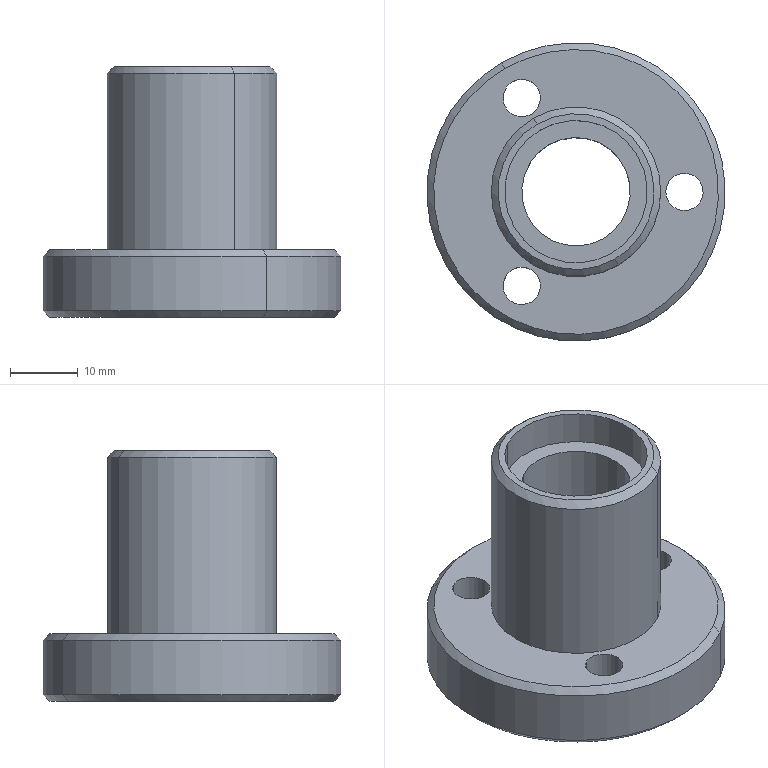Component | SolidWorks | JYTBJ-HeaderPlateFlangeSeatB-1 | 1 solid | 36 faces | box 44 x 44 x 37 mm | volume 17743 mm3 | cylinder 22 | plane 8 | cone 6 | commonest cylinder face diameters 10 x6 5.5 x6 21 x4 25 x2 16 x2 44 x2
STEP:
#1=COLOUR_RGB('',0.7922,0.8196,0.9333);
#2=FILL_AREA_STYLE_COLOUR('',#1);
#3=FILL_AREA_STYLE('',(#2));
#4=SURFACE_STYLE_FILL_AREA(#3);
#5=SURFACE_SIDE_STYLE('',(#4));
#6=SURFACE_STYLE_USAGE(.BOTH.,#5);
#7=PRESENTATION_STYLE_ASSIGNMENT((#6));
#8=CARTESIAN_POINT('',(-3.046,9.321,-0.03937));
#9=VERTEX_POINT('',#8);
#10=CARTESIAN_POINT('',(-2.594,8.536,-0.03937));
#11=VERTEX_POINT('',#10);
#12=CARTESIAN_POINT('',(-2.82,8.928,-0.03937));
#13=DIRECTION('',(0.,0.,1.));
#14=DIRECTION('',(-0.5,0.866,0.));
#15=AXIS2_PLACEMENT_3D('',#12,#13,#14);
#16=CIRCLE('',#15,0.4528);
#17=EDGE_CURVE('',#9,#11,#16,.T.);
#18=ORIENTED_EDGE('',*,*,#17,.F.);
#19=CARTESIAN_POINT('',(-3.066,9.355,-0.07874));
#20=VERTEX_POINT('',#19);
#21=CARTESIAN_POINT('',(-3.066,9.355,-0.07874));
#22=DIRECTION('',(-0.3536,0.6124,-0.7071));
#23=VECTOR('',#22,39.37);
#24=LINE('',#21,#23);
#25=EDGE_CURVE('',#9,#20,#24,.T.);
#26=ORIENTED_EDGE('',*,*,#25,.T.);
#27=CARTESIAN_POINT('',(-2.574,8.502,-0.07874));
#28=VERTEX_POINT('',#27);
#29=CARTESIAN_POINT('',(-2.82,8.928,-0.07874));
#30=DIRECTION('',(0.,0.,-1.));
#31=DIRECTION('',(-0.5,0.866,0.));
#32=AXIS2_PLACEMENT_3D('',#29,#30,#31);
#33=CIRCLE('',#32,0.4921);
#34=EDGE_CURVE('',#28,#20,#33,.T.);
#35=ORIENTED_EDGE('',*,*,#34,.F.);
#36=CARTESIAN_POINT('',(-2.574,8.502,-0.07874));
#37=DIRECTION('',(0.3536,-0.6124,-0.7071));
#38=VECTOR('',#37,39.37);
#39=LINE('',#36,#38);
#40=EDGE_CURVE('',#11,#28,#39,.T.);
#41=ORIENTED_EDGE('',*,*,#40,.F.);
#42=EDGE_LOOP('',(#18,#26,#35,#41));
#43=FACE_OUTER_BOUND('',#42,.T.);
#44=CARTESIAN_POINT('',(-2.82,8.928,-0.07874));
#45=DIRECTION('',(0.,0.,-1.));
#46=DIRECTION('',(0.5,-0.866,0.));
#47=AXIS2_PLACEMENT_3D('',#44,#45,#46);
#48=CONICAL_SURFACE('',#47,0.4921,0.7854);
#49=ADVANCED_FACE('',(#43),#48,.T.);
#50=CARTESIAN_POINT('',(-3.233,9.644,-1.102));
#51=VERTEX_POINT('',#50);
#52=CARTESIAN_POINT('',(-2.407,8.212,-1.102));
#53=VERTEX_POINT('',#52);
#54=CARTESIAN_POINT('',(-2.82,8.928,-1.102));
#55=DIRECTION('',(0.,0.,1.));
#56=DIRECTION('',(-0.5,0.866,0.));
#57=AXIS2_PLACEMENT_3D('',#54,#55,#56);
#58=CIRCLE('',#57,0.8268);
#59=EDGE_CURVE('',#51,#53,#58,.T.);
#60=ORIENTED_EDGE('',*,*,#59,.F.);
#61=CARTESIAN_POINT('',(-3.253,9.679,-1.142));
#62=VERTEX_POINT('',#61);
#63=CARTESIAN_POINT('',(-3.253,9.679,-1.142));
#64=DIRECTION('',(-0.3536,0.6124,-0.7071));
#65=VECTOR('',#64,39.37);
#66=LINE('',#63,#65);
#67=EDGE_CURVE('',#51,#62,#66,.T.);
#68=ORIENTED_EDGE('',*,*,#67,.T.);
#69=CARTESIAN_POINT('',(-2.387,8.178,-1.142));
#70=VERTEX_POINT('',#69);
#71=CARTESIAN_POINT('',(-2.82,8.928,-1.142));
#72=DIRECTION('',(0.,0.,-1.));
#73=DIRECTION('',(-0.5,0.866,0.));
#74=AXIS2_PLACEMENT_3D('',#71,#72,#73);
#75=CIRCLE('',#74,0.8661);
#76=EDGE_CURVE('',#70,#62,#75,.T.);
#77=ORIENTED_EDGE('',*,*,#76,.F.);
#78=CARTESIAN_POINT('',(-2.387,8.178,-1.142));
#79=DIRECTION('',(0.3536,-0.6124,-0.7071));
#80=VECTOR('',#79,39.37);
#81=LINE('',#78,#80);
#82=EDGE_CURVE('',#53,#70,#81,.T.);
#83=ORIENTED_EDGE('',*,*,#82,.F.);
#84=EDGE_LOOP('',(#60,#68,#77,#83));
#85=FACE_OUTER_BOUND('',#84,.T.);
#86=CARTESIAN_POINT('',(-2.82,8.928,-1.142));
#87=DIRECTION('',(0.,0.,-1.));
#88=DIRECTION('',(0.5,-0.866,0.));
#89=AXIS2_PLACEMENT_3D('',#86,#87,#88);
#90=CONICAL_SURFACE('',#89,0.8661,0.7854);
#91=ADVANCED_FACE('',(#85),#90,.T.);
#92=CARTESIAN_POINT('',(-2.407,8.212,-1.496));
#93=VERTEX_POINT('',#92);
#94=CARTESIAN_POINT('',(-3.233,8.212,-1.496));
#95=VERTEX_POINT('',#94);
#96=CARTESIAN_POINT('',(-2.82,8.928,-1.496));
#97=DIRECTION('',(0.,0.,-1.));
#98=DIRECTION('',(0.5,-0.866,0.));
#99=AXIS2_PLACEMENT_3D('',#96,#97,#98);
#100=CIRCLE('',#99,0.8268);
#101=EDGE_CURVE('',#93,#95,#100,.T.);
#102=ORIENTED_EDGE('',*,*,#101,.F.);
#103=CARTESIAN_POINT('',(-2.387,8.178,-1.457));
#104=VERTEX_POINT('',#103);
#105=CARTESIAN_POINT('',(-2.407,8.212,-1.496));
#106=DIRECTION('',(0.3536,-0.6124,0.7071));
#107=VECTOR('',#106,39.37);
#108=LINE('',#105,#107);
#109=EDGE_CURVE('',#93,#104,#108,.T.);
#110=ORIENTED_EDGE('',*,*,#109,.T.);
#111=CARTESIAN_POINT('',(-3.253,9.679,-1.457));
#112=VERTEX_POINT('',#111);
#113=CARTESIAN_POINT('',(-2.82,8.928,-1.457));
#114=DIRECTION('',(0.,0.,1.));
#115=DIRECTION('',(0.5,-0.866,0.));
#116=AXIS2_PLACEMENT_3D('',#113,#114,#115);
#117=CIRCLE('',#116,0.8661);
#118=EDGE_CURVE('',#112,#104,#117,.T.);
#119=ORIENTED_EDGE('',*,*,#118,.F.);
#120=CARTESIAN_POINT('',(-3.233,9.644,-1.496));
#121=VERTEX_POINT('',#120);
#122=CARTESIAN_POINT('',(-3.233,9.644,-1.496));
#123=DIRECTION('',(-0.3536,0.6124,0.7071));
#124=VECTOR('',#123,39.37);
#125=LINE('',#122,#124);
#126=EDGE_CURVE('',#121,#112,#125,.T.);
#127=ORIENTED_EDGE('',*,*,#126,.F.);
#128=CARTESIAN_POINT('',(-2.82,8.928,-1.496));
#129=DIRECTION('',(0.,0.,-1.));
#130=DIRECTION('',(0.5,-0.866,0.));
#131=AXIS2_PLACEMENT_3D('',#128,#129,#130);
#132=CIRCLE('',#131,0.8268);
#133=EDGE_CURVE('',#95,#121,#132,.T.);
#134=ORIENTED_EDGE('',*,*,#133,.F.);
#135=EDGE_LOOP('',(#102,#110,#119,#127,#134));
#136=FACE_OUTER_BOUND('',#135,.T.);
#137=CARTESIAN_POINT('',(-2.82,8.928,-1.496));
#138=DIRECTION('',(0.,0.,1.));
#139=DIRECTION('',(-0.5,0.866,0.));
#140=AXIS2_PLACEMENT_3D('',#137,#138,#139);
#141=CONICAL_SURFACE('',#140,0.8268,0.7854);
#142=ADVANCED_FACE('',(#136),#141,.T.);
#143=CARTESIAN_POINT('',(-3.233,8.553,-1.272));
#144=VERTEX_POINT('',#143);
#145=CARTESIAN_POINT('',(-3.036,8.212,-1.272));
#146=VERTEX_POINT('',#145);
#147=CARTESIAN_POINT('',(-3.135,8.383,-1.272));
#148=DIRECTION('',(0.,0.,-1.));
#149=DIRECTION('',(0.5,-0.866,0.));
#150=AXIS2_PLACEMENT_3D('',#147,#148,#149);
#151=CIRCLE('',#150,0.1969);
#152=EDGE_CURVE('',#144,#146,#151,.T.);
#153=ORIENTED_EDGE('',*,*,#152,.F.);
#154=CARTESIAN_POINT('',(-3.233,8.553,-1.496));
#155=VERTEX_POINT('',#154);
#156=CARTESIAN_POINT('',(-3.233,8.553,-1.496));
#157=DIRECTION('',(0.,0.,-1.));
#158=VECTOR('',#157,39.37);
#159=LINE('',#156,#158);
#160=EDGE_CURVE('',#144,#155,#159,.T.);
#161=ORIENTED_EDGE('',*,*,#160,.T.);
#162=CARTESIAN_POINT('',(-3.036,8.212,-1.496));
#163=VERTEX_POINT('',#162);
#164=CARTESIAN_POINT('',(-3.135,8.383,-1.496));
#165=DIRECTION('',(0.,0.,-1.));
#166=DIRECTION('',(0.5,-0.866,0.));
#167=AXIS2_PLACEMENT_3D('',#164,#165,#166);
#168=CIRCLE('',#167,0.1969);
#169=EDGE_CURVE('',#155,#163,#168,.T.);
#170=ORIENTED_EDGE('',*,*,#169,.T.);
#171=CARTESIAN_POINT('',(-3.036,8.212,-1.496));
#172=DIRECTION('',(0.,0.,-1.));
#173=VECTOR('',#172,39.37);
#174=LINE('',#171,#173);
#175=EDGE_CURVE('',#146,#163,#174,.T.);
#176=ORIENTED_EDGE('',*,*,#175,.F.);
#177=EDGE_LOOP('',(#153,#161,#170,#176));
#178=FACE_OUTER_BOUND('',#177,.T.);
#179=CARTESIAN_POINT('',(-3.135,8.383,-1.496));
#180=DIRECTION('',(0.,0.,-1.));
#181=DIRECTION('',(0.5,-0.866,0.));
#182=AXIS2_PLACEMENT_3D('',#179,#180,#181);
#183=CYLINDRICAL_SURFACE('',#182,0.1969);
#184=ADVANCED_FACE('',(#178),#183,.F.);
#185=CARTESIAN_POINT('',(-3.081,8.289,-1.102));
#186=VERTEX_POINT('',#185);
#187=CARTESIAN_POINT('',(-3.189,8.477,-1.102));
#188=VERTEX_POINT('',#187);
#189=CARTESIAN_POINT('',(-3.135,8.383,-1.102));
#190=DIRECTION('',(0.,0.,1.));
#191=DIRECTION('',(-0.5,0.866,0.));
#192=AXIS2_PLACEMENT_3D('',#189,#190,#191);
#193=CIRCLE('',#192,0.1083);
#194=EDGE_CURVE('',#186,#188,#193,.T.);
#195=ORIENTED_EDGE('',*,*,#194,.T.);
#196=CARTESIAN_POINT('',(-3.189,8.477,-1.272));
#197=VERTEX_POINT('',#196);
#198=CARTESIAN_POINT('',(-3.189,8.477,-1.496));
#199=DIRECTION('',(0.,0.,-1.));
#200=VECTOR('',#199,39.37);
#201=LINE('',#198,#200);
#202=EDGE_CURVE('',#188,#197,#201,.T.);
#203=ORIENTED_EDGE('',*,*,#202,.T.);
#204=CARTESIAN_POINT('',(-3.081,8.289,-1.272));
#205=VERTEX_POINT('',#204);
#206=CARTESIAN_POINT('',(-3.135,8.383,-1.272));
#207=DIRECTION('',(0.,0.,-1.));
#208=DIRECTION('',(0.5,-0.866,0.));
#209=AXIS2_PLACEMENT_3D('',#206,#207,#208);
#210=CIRCLE('',#209,0.1083);
#211=EDGE_CURVE('',#197,#205,#210,.T.);
#212=ORIENTED_EDGE('',*,*,#211,.T.);
#213=CARTESIAN_POINT('',(-3.081,8.289,-1.496));
#214=DIRECTION('',(0.,0.,-1.));
#215=VECTOR('',#214,39.37);
#216=LINE('',#213,#215);
#217=EDGE_CURVE('',#186,#205,#216,.T.);
#218=ORIENTED_EDGE('',*,*,#217,.F.);
#219=EDGE_LOOP('',(#195,#203,#212,#218));
#220=FACE_OUTER_BOUND('',#219,.T.);
#221=CARTESIAN_POINT('',(-3.135,8.383,-1.496));
#222=DIRECTION('',(0.,0.,-1.));
#223=DIRECTION('',(0.5,-0.866,0.));
#224=AXIS2_PLACEMENT_3D('',#221,#222,#223);
#225=CYLINDRICAL_SURFACE('',#224,0.1083);
#226=ADVANCED_FACE('',(#220),#225,.F.);
#227=CARTESIAN_POINT('',(-2.288,9.099,-1.272));
#228=VERTEX_POINT('',#227);
#229=CARTESIAN_POINT('',(-2.092,8.758,-1.272));
#230=VERTEX_POINT('',#229);
#231=CARTESIAN_POINT('',(-2.19,8.928,-1.272));
#232=DIRECTION('',(0.,0.,-1.));
#233=DIRECTION('',(0.5,-0.866,0.));
#234=AXIS2_PLACEMENT_3D('',#231,#232,#233);
#235=CIRCLE('',#234,0.1969);
#236=EDGE_CURVE('',#228,#230,#235,.T.);
#237=ORIENTED_EDGE('',*,*,#236,.F.);
#238=CARTESIAN_POINT('',(-2.288,9.099,-1.496));
#239=VERTEX_POINT('',#238);
#240=CARTESIAN_POINT('',(-2.288,9.099,-1.496));
#241=DIRECTION('',(0.,0.,-1.));
#242=VECTOR('',#241,39.37);
#243=LINE('',#240,#242);
#244=EDGE_CURVE('',#228,#239,#243,.T.);
#245=ORIENTED_EDGE('',*,*,#244,.T.);
#246=CARTESIAN_POINT('',(-1.993,8.928,-1.496));
#247=VERTEX_POINT('',#246);
#248=CARTESIAN_POINT('',(-2.19,8.928,-1.496));
#249=DIRECTION('',(0.,0.,-1.));
#250=DIRECTION('',(0.5,-0.866,0.));
#251=AXIS2_PLACEMENT_3D('',#248,#249,#250);
#252=CIRCLE('',#251,0.1969);
#253=EDGE_CURVE('',#239,#247,#252,.T.);
#254=ORIENTED_EDGE('',*,*,#253,.T.);
#255=CARTESIAN_POINT('',(-2.092,8.758,-1.496));
#256=VERTEX_POINT('',#255);
#257=CARTESIAN_POINT('',(-2.19,8.928,-1.496));
#258=DIRECTION('',(0.,0.,-1.));
#259=DIRECTION('',(0.5,-0.866,0.));
#260=AXIS2_PLACEMENT_3D('',#257,#258,#259);
#261=CIRCLE('',#260,0.1969);
#262=EDGE_CURVE('',#247,#256,#261,.T.);
#263=ORIENTED_EDGE('',*,*,#262,.T.);
#264=CARTESIAN_POINT('',(-2.092,8.758,-1.496));
#265=DIRECTION('',(0.,0.,-1.));
#266=VECTOR('',#265,39.37);
#267=LINE('',#264,#266);
#268=EDGE_CURVE('',#230,#256,#267,.T.);
#269=ORIENTED_EDGE('',*,*,#268,.F.);
#270=EDGE_LOOP('',(#237,#245,#254,#263,#269));
#271=FACE_OUTER_BOUND('',#270,.T.);
#272=CARTESIAN_POINT('',(-2.19,8.928,-1.496));
#273=DIRECTION('',(0.,0.,-1.));
#274=DIRECTION('',(0.5,-0.866,0.));
#275=AXIS2_PLACEMENT_3D('',#272,#273,#274);
#276=CYLINDRICAL_SURFACE('',#275,0.1969);
#277=ADVANCED_FACE('',(#271),#276,.F.);
#278=CARTESIAN_POINT('',(-2.136,8.835,-1.102));
#279=VERTEX_POINT('',#278);
#280=CARTESIAN_POINT('',(-2.244,9.022,-1.102));
#281=VERTEX_POINT('',#280);
#282=CARTESIAN_POINT('',(-2.19,8.928,-1.102));
#283=DIRECTION('',(0.,0.,1.));
#284=DIRECTION('',(-0.5,0.866,0.));
#285=AXIS2_PLACEMENT_3D('',#282,#283,#284);
#286=CIRCLE('',#285,0.1083);
#287=EDGE_CURVE('',#279,#281,#286,.T.);
#288=ORIENTED_EDGE('',*,*,#287,.T.);
#289=CARTESIAN_POINT('',(-2.244,9.022,-1.272));
#290=VERTEX_POINT('',#289);
#291=CARTESIAN_POINT('',(-2.244,9.022,-1.496));
#292=DIRECTION('',(0.,0.,-1.));
#293=VECTOR('',#292,39.37);
#294=LINE('',#291,#293);
#295=EDGE_CURVE('',#281,#290,#294,.T.);
#296=ORIENTED_EDGE('',*,*,#295,.T.);
#297=CARTESIAN_POINT('',(-2.136,8.835,-1.272));
#298=VERTEX_POINT('',#297);
#299=CARTESIAN_POINT('',(-2.19,8.928,-1.272));
#300=DIRECTION('',(0.,0.,-1.));
#301=DIRECTION('',(0.5,-0.866,0.));
#302=AXIS2_PLACEMENT_3D('',#299,#300,#301);
#303=CIRCLE('',#302,0.1083);
#304=EDGE_CURVE('',#290,#298,#303,.T.);
#305=ORIENTED_EDGE('',*,*,#304,.T.);
#306=CARTESIAN_POINT('',(-2.136,8.835,-1.496));
#307=DIRECTION('',(0.,0.,-1.));
#308=VECTOR('',#307,39.37);
#309=LINE('',#306,#308);
#310=EDGE_CURVE('',#279,#298,#309,.T.);
#311=ORIENTED_EDGE('',*,*,#310,.F.);
#312=EDGE_LOOP('',(#288,#296,#305,#311));
#313=FACE_OUTER_BOUND('',#312,.T.);
#314=CARTESIAN_POINT('',(-2.19,8.928,-1.496));
#315=DIRECTION('',(0.,0.,-1.));
#316=DIRECTION('',(0.5,-0.866,0.));
#317=AXIS2_PLACEMENT_3D('',#314,#315,#316);
#318=CYLINDRICAL_SURFACE('',#317,0.1083);
#319=ADVANCED_FACE('',(#313),#318,.F.);
#320=CARTESIAN_POINT('',(-3.233,9.644,-1.272));
#321=VERTEX_POINT('',#320);
#322=CARTESIAN_POINT('',(-3.036,9.303,-1.272));
#323=VERTEX_POINT('',#322);
#324=CARTESIAN_POINT('',(-3.135,9.474,-1.272));
#325=DIRECTION('',(0.,0.,-1.));
#326=DIRECTION('',(0.5,-0.866,0.));
#327=AXIS2_PLACEMENT_3D('',#324,#325,#326);
#328=CIRCLE('',#327,0.1969);
#329=EDGE_CURVE('',#321,#323,#328,.T.);
#330=ORIENTED_EDGE('',*,*,#329,.F.);
#331=CARTESIAN_POINT('',(-3.233,9.644,-1.496));
#332=DIRECTION('',(0.,0.,-1.));
#333=VECTOR('',#332,39.37);
#334=LINE('',#331,#333);
#335=EDGE_CURVE('',#321,#121,#334,.T.);
#336=ORIENTED_EDGE('',*,*,#335,.T.);
#337=CARTESIAN_POINT('',(-3.036,9.303,-1.496));
#338=VERTEX_POINT('',#337);
#339=CARTESIAN_POINT('',(-3.135,9.474,-1.496));
#340=DIRECTION('',(0.,0.,-1.));
#341=DIRECTION('',(0.5,-0.866,0.));
#342=AXIS2_PLACEMENT_3D('',#339,#340,#341);
#343=CIRCLE('',#342,0.1969);
#344=EDGE_CURVE('',#121,#338,#343,.T.);
#345=ORIENTED_EDGE('',*,*,#344,.T.);
#346=CARTESIAN_POINT('',(-3.036,9.303,-1.496));
#347=DIRECTION('',(0.,0.,-1.));
#348=VECTOR('',#347,39.37);
#349=LINE('',#346,#348);
#350=EDGE_CURVE('',#323,#338,#349,.T.);
#351=ORIENTED_EDGE('',*,*,#350,.F.);
#352=EDGE_LOOP('',(#330,#336,#345,#351));
#353=FACE_OUTER_BOUND('',#352,.T.);
#354=CARTESIAN_POINT('',(-3.135,9.474,-1.496));
#355=DIRECTION('',(0.,0.,-1.));
#356=DIRECTION('',(0.5,-0.866,0.));
#357=AXIS2_PLACEMENT_3D('',#354,#355,#356);
#358=CYLINDRICAL_SURFACE('',#357,0.1969);
#359=ADVANCED_FACE('',(#353),#358,.F.);
#360=CARTESIAN_POINT('',(-3.081,9.38,-1.102));
#361=VERTEX_POINT('',#360);
#362=CARTESIAN_POINT('',(-3.189,9.568,-1.102));
#363=VERTEX_POINT('',#362);
#364=CARTESIAN_POINT('',(-3.135,9.474,-1.102));
#365=DIRECTION('',(0.,0.,1.));
#366=DIRECTION('',(-0.5,0.866,0.));
#367=AXIS2_PLACEMENT_3D('',#364,#365,#366);
#368=CIRCLE('',#367,0.1083);
#369=EDGE_CURVE('',#361,#363,#368,.T.);
#370=ORIENTED_EDGE('',*,*,#369,.T.);
#371=CARTESIAN_POINT('',(-3.189,9.568,-1.272));
#372=VERTEX_POINT('',#371);
#373=CARTESIAN_POINT('',(-3.189,9.568,-1.496));
#374=DIRECTION('',(0.,0.,-1.));
#375=VECTOR('',#374,39.37);
#376=LINE('',#373,#375);
#377=EDGE_CURVE('',#363,#372,#376,.T.);
#378=ORIENTED_EDGE('',*,*,#377,.T.);
#379=CARTESIAN_POINT('',(-3.081,9.38,-1.272));
#380=VERTEX_POINT('',#379);
#381=CARTESIAN_POINT('',(-3.135,9.474,-1.272));
#382=DIRECTION('',(0.,0.,-1.));
#383=DIRECTION('',(0.5,-0.866,0.));
#384=AXIS2_PLACEMENT_3D('',#381,#382,#383);
#385=CIRCLE('',#384,0.1083);
#386=EDGE_CURVE('',#372,#380,#385,.T.);
#387=ORIENTED_EDGE('',*,*,#386,.T.);
#388=CARTESIAN_POINT('',(-3.081,9.38,-1.496));
#389=DIRECTION('',(0.,0.,-1.));
#390=VECTOR('',#389,39.37);
#391=LINE('',#388,#390);
#392=EDGE_CURVE('',#361,#380,#391,.T.);
#393=ORIENTED_EDGE('',*,*,#392,.F.);
#394=EDGE_LOOP('',(#370,#378,#387,#393));
#395=FACE_OUTER_BOUND('',#394,.T.);
#396=CARTESIAN_POINT('',(-3.135,9.474,-1.496));
#397=DIRECTION('',(0.,0.,-1.));
#398=DIRECTION('',(0.5,-0.866,0.));
#399=AXIS2_PLACEMENT_3D('',#396,#397,#398);
#400=CYLINDRICAL_SURFACE('',#399,0.1083);
#401=ADVANCED_FACE('',(#395),#400,.F.);
#402=ORIENTED_EDGE('',*,*,#34,.T.);
#403=CARTESIAN_POINT('',(-3.066,9.355,-1.102));
#404=VERTEX_POINT('',#403);
#405=CARTESIAN_POINT('',(-3.066,9.355,-1.358));
#406=DIRECTION('',(0.,0.,-1.));
#407=VECTOR('',#406,39.37);
#408=LINE('',#405,#407);
#409=EDGE_CURVE('',#20,#404,#408,.T.);
#410=ORIENTED_EDGE('',*,*,#409,.T.);
#411=CARTESIAN_POINT('',(-2.574,8.502,-1.102));
#412=VERTEX_POINT('',#411);
#413=CARTESIAN_POINT('',(-2.82,8.928,-1.102));
#414=DIRECTION('',(0.,0.,-1.));
#415=DIRECTION('',(0.5,-0.866,0.));
#416=AXIS2_PLACEMENT_3D('',#413,#414,#415);
#417=CIRCLE('',#416,0.4921);
#418=EDGE_CURVE('',#412,#404,#417,.T.);
#419=ORIENTED_EDGE('',*,*,#418,.F.);
#420=CARTESIAN_POINT('',(-2.574,8.502,-1.358));
#421=DIRECTION('',(0.,0.,-1.));
#422=VECTOR('',#421,39.37);
#423=LINE('',#420,#422);
#424=EDGE_CURVE('',#28,#412,#423,.T.);
#425=ORIENTED_EDGE('',*,*,#424,.F.);
#426=EDGE_LOOP('',(#402,#410,#419,#425));
#427=FACE_OUTER_BOUND('',#426,.T.);
#428=CARTESIAN_POINT('',(-2.82,8.928,-1.358));
#429=DIRECTION('',(0.,0.,-1.));
#430=DIRECTION('',(0.5,-0.866,0.));
#431=AXIS2_PLACEMENT_3D('',#428,#429,#430);
#432=CYLINDRICAL_SURFACE('',#431,0.4921);
#433=ADVANCED_FACE('',(#427),#432,.T.);
#434=CARTESIAN_POINT('',(-3.027,9.286,-0.03937));
#435=VERTEX_POINT('',#434);
#436=CARTESIAN_POINT('',(-2.613,8.57,-0.03937));
#437=VERTEX_POINT('',#436);
#438=CARTESIAN_POINT('',(-2.82,8.928,-0.03937));
#439=DIRECTION('',(0.,0.,-1.));
#440=DIRECTION('',(0.5,-0.866,0.));
#441=AXIS2_PLACEMENT_3D('',#438,#439,#440);
#442=CIRCLE('',#441,0.4134);
#443=EDGE_CURVE('',#435,#437,#442,.T.);
#444=ORIENTED_EDGE('',*,*,#443,.F.);
#445=CARTESIAN_POINT('',(-3.027,9.286,-0.2362));
#446=VERTEX_POINT('',#445);
#447=CARTESIAN_POINT('',(-3.027,9.286,-1.358));
#448=DIRECTION('',(0.,0.,-1.));
#449=VECTOR('',#448,39.37);
#450=LINE('',#447,#449);
#451=EDGE_CURVE('',#435,#446,#450,.T.);
#452=ORIENTED_EDGE('',*,*,#451,.T.);
#453=CARTESIAN_POINT('',(-2.613,8.57,-0.2362));
#454=VERTEX_POINT('',#453);
#455=CARTESIAN_POINT('',(-2.82,8.928,-0.2362));
#456=DIRECTION('',(0.,0.,-1.));
#457=DIRECTION('',(0.5,-0.866,0.));
#458=AXIS2_PLACEMENT_3D('',#455,#456,#457);
#459=CIRCLE('',#458,0.4134);
#460=EDGE_CURVE('',#446,#454,#459,.T.);
#461=ORIENTED_EDGE('',*,*,#460,.T.);
#462=CARTESIAN_POINT('',(-2.613,8.57,-1.358));
#463=DIRECTION('',(0.,0.,-1.));
#464=VECTOR('',#463,39.37);
#465=LINE('',#462,#464);
#466=EDGE_CURVE('',#437,#454,#465,.T.);
#467=ORIENTED_EDGE('',*,*,#466,.F.);
#468=EDGE_LOOP('',(#444,#452,#461,#467));
#469=FACE_OUTER_BOUND('',#468,.T.);
#470=CARTESIAN_POINT('',(-2.82,8.928,-1.358));
#471=DIRECTION('',(0.,0.,-1.));
#472=DIRECTION('',(0.5,-0.866,0.));
#473=AXIS2_PLACEMENT_3D('',#470,#471,#472);
#474=CYLINDRICAL_SURFACE('',#473,0.4134);
#475=ADVANCED_FACE('',(#469),#474,.F.);
#476=CARTESIAN_POINT('',(-2.977,9.201,-0.2362));
#477=VERTEX_POINT('',#476);
#478=CARTESIAN_POINT('',(-2.662,8.656,-0.2362));
#479=VERTEX_POINT('',#478);
#480=CARTESIAN_POINT('',(-2.82,8.928,-0.2362));
#481=DIRECTION('',(0.,0.,-1.));
#482=DIRECTION('',(0.5,-0.866,0.));
#483=AXIS2_PLACEMENT_3D('',#480,#481,#482);
#484=CIRCLE('',#483,0.315);
#485=EDGE_CURVE('',#477,#479,#484,.T.);
#486=ORIENTED_EDGE('',*,*,#485,.F.);
#487=CARTESIAN_POINT('',(-2.977,9.201,-1.299));
#488=VERTEX_POINT('',#487);
#489=CARTESIAN_POINT('',(-2.977,9.201,-1.358));
#490=DIRECTION('',(0.,0.,-1.));
#491=VECTOR('',#490,39.37);
#492=LINE('',#489,#491);
#493=EDGE_CURVE('',#477,#488,#492,.T.);
#494=ORIENTED_EDGE('',*,*,#493,.T.);
#495=CARTESIAN_POINT('',(-2.662,8.656,-1.299));
#496=VERTEX_POINT('',#495);
#497=CARTESIAN_POINT('',(-2.82,8.928,-1.299));
#498=DIRECTION('',(0.,0.,-1.));
#499=DIRECTION('',(0.5,-0.866,0.));
#500=AXIS2_PLACEMENT_3D('',#497,#498,#499);
#501=CIRCLE('',#500,0.315);
#502=EDGE_CURVE('',#488,#496,#501,.T.);
#503=ORIENTED_EDGE('',*,*,#502,.T.);
#504=CARTESIAN_POINT('',(-2.662,8.656,-1.358));
#505=DIRECTION('',(0.,0.,-1.));
#506=VECTOR('',#505,39.37);
#507=LINE('',#504,#506);
#508=EDGE_CURVE('',#479,#496,#507,.T.);
#509=ORIENTED_EDGE('',*,*,#508,.F.);
#510=EDGE_LOOP('',(#486,#494,#503,#509));
#511=FACE_OUTER_BOUND('',#510,.T.);
#512=CARTESIAN_POINT('',(-2.82,8.928,-1.358));
#513=DIRECTION('',(0.,0.,-1.));
#514=DIRECTION('',(0.5,-0.866,0.));
#515=AXIS2_PLACEMENT_3D('',#512,#513,#514);
#516=CYLINDRICAL_SURFACE('',#515,0.315);
#517=ADVANCED_FACE('',(#511),#516,.F.);
#518=CARTESIAN_POINT('',(-3.027,9.286,-1.299));
#519=VERTEX_POINT('',#518);
#520=CARTESIAN_POINT('',(-2.613,8.57,-1.299));
#521=VERTEX_POINT('',#520);
#522=CARTESIAN_POINT('',(-2.82,8.928,-1.299));
#523=DIRECTION('',(0.,0.,-1.));
#524=DIRECTION('',(0.5,-0.866,0.));
#525=AXIS2_PLACEMENT_3D('',#522,#523,#524);
#526=CIRCLE('',#525,0.4134);
#527=EDGE_CURVE('',#519,#521,#526,.T.);
#528=ORIENTED_EDGE('',*,*,#527,.F.);
#529=CARTESIAN_POINT('',(-3.027,9.286,-1.496));
#530=VERTEX_POINT('',#529);
#531=CARTESIAN_POINT('',(-3.027,9.286,-1.358));
#532=DIRECTION('',(0.,0.,-1.));
#533=VECTOR('',#532,39.37);
#534=LINE('',#531,#533);
#535=EDGE_CURVE('',#519,#530,#534,.T.);
#536=ORIENTED_EDGE('',*,*,#535,.T.);
#537=CARTESIAN_POINT('',(-2.613,8.57,-1.496));
#538=VERTEX_POINT('',#537);
#539=CARTESIAN_POINT('',(-2.82,8.928,-1.496));
#540=DIRECTION('',(0.,0.,-1.));
#541=DIRECTION('',(0.5,-0.866,0.));
#542=AXIS2_PLACEMENT_3D('',#539,#540,#541);
#543=CIRCLE('',#542,0.4134);
#544=EDGE_CURVE('',#530,#538,#543,.T.);
#545=ORIENTED_EDGE('',*,*,#544,.T.);
#546=CARTESIAN_POINT('',(-2.613,8.57,-1.358));
#547=DIRECTION('',(0.,0.,-1.));
#548=VECTOR('',#547,39.37);
#549=LINE('',#546,#548);
#550=EDGE_CURVE('',#521,#538,#549,.T.);
#551=ORIENTED_EDGE('',*,*,#550,.F.);
#552=EDGE_LOOP('',(#528,#536,#545,#551));
#553=FACE_OUTER_BOUND('',#552,.T.);
#554=CARTESIAN_POINT('',(-2.82,8.928,-1.358));
#555=DIRECTION('',(0.,0.,-1.));
#556=DIRECTION('',(0.5,-0.866,0.));
#557=AXIS2_PLACEMENT_3D('',#554,#555,#556);
#558=CYLINDRICAL_SURFACE('',#557,0.4134);
#559=ADVANCED_FACE('',(#553),#558,.F.);
#560=ORIENTED_EDGE('',*,*,#76,.T.);
#561=CARTESIAN_POINT('',(-3.253,9.679,-1.358));
#562=DIRECTION('',(0.,0.,-1.));
#563=VECTOR('',#562,39.37);
#564=LINE('',#561,#563);
#565=EDGE_CURVE('',#62,#112,#564,.T.);
#566=ORIENTED_EDGE('',*,*,#565,.T.);
#567=ORIENTED_EDGE('',*,*,#118,.T.);
#568=CARTESIAN_POINT('',(-2.387,8.178,-1.358));
#569=DIRECTION('',(0.,0.,-1.));
#570=VECTOR('',#569,39.37);
#571=LINE('',#568,#570);
#572=EDGE_CURVE('',#70,#104,#571,.T.);
#573=ORIENTED_EDGE('',*,*,#572,.F.);
#574=EDGE_LOOP('',(#560,#566,#567,#573));
#575=FACE_OUTER_BOUND('',#574,.T.);
#576=CARTESIAN_POINT('',(-2.82,8.928,-1.358));
#577=DIRECTION('',(0.,0.,-1.));
#578=DIRECTION('',(0.5,-0.866,0.));
#579=AXIS2_PLACEMENT_3D('',#576,#577,#578);
#580=CYLINDRICAL_SURFACE('',#579,0.8661);
#581=ADVANCED_FACE('',(#575),#580,.T.);
#582=ORIENTED_EDGE('',*,*,#565,.F.);
#583=CARTESIAN_POINT('',(-2.82,8.928,-1.142));
#584=DIRECTION('',(0.,0.,-1.));
#585=DIRECTION('',(-0.5,0.866,0.));
#586=AXIS2_PLACEMENT_3D('',#583,#584,#585);
#587=CIRCLE('',#586,0.8661);
#588=EDGE_CURVE('',#62,#70,#587,.T.);
#589=ORIENTED_EDGE('',*,*,#588,.T.);
#590=ORIENTED_EDGE('',*,*,#572,.T.);
#591=CARTESIAN_POINT('',(-2.82,8.928,-1.457));
#592=DIRECTION('',(0.,0.,1.));
#593=DIRECTION('',(0.5,-0.866,0.));
#594=AXIS2_PLACEMENT_3D('',#591,#592,#593);
#595=CIRCLE('',#594,0.8661);
#596=EDGE_CURVE('',#104,#112,#595,.T.);
#597=ORIENTED_EDGE('',*,*,#596,.T.);
#598=EDGE_LOOP('',(#582,#589,#590,#597));
#599=FACE_OUTER_BOUND('',#598,.T.);
#600=CARTESIAN_POINT('',(-2.82,8.928,-1.358));
#601=DIRECTION('',(0.,0.,-1.));
#602=DIRECTION('',(0.5,-0.866,0.));
#603=AXIS2_PLACEMENT_3D('',#600,#601,#602);
#604=CYLINDRICAL_SURFACE('',#603,0.8661);
#605=ADVANCED_FACE('',(#599),#604,.T.);
#606=CARTESIAN_POINT('',(-3.135,8.383,-1.496));
#607=DIRECTION('',(0.,0.,-1.));
#608=DIRECTION('',(0.5,-0.866,0.));
#609=AXIS2_PLACEMENT_3D('',#606,#607,#608);
#610=CIRCLE('',#609,0.1969);
#611=EDGE_CURVE('',#95,#155,#610,.T.);
#612=ORIENTED_EDGE('',*,*,#611,.F.);
#613=ORIENTED_EDGE('',*,*,#133,.T.);
#614=CARTESIAN_POINT('',(-3.135,9.474,-1.496));
#615=DIRECTION('',(0.,0.,-1.));
#616=DIRECTION('',(0.5,-0.866,0.));
#617=AXIS2_PLACEMENT_3D('',#614,#615,#616);
#618=CIRCLE('',#617,0.1969);
#619=EDGE_CURVE('',#338,#121,#618,.T.);
#620=ORIENTED_EDGE('',*,*,#619,.F.);
#621=ORIENTED_EDGE('',*,*,#344,.F.);
#622=CARTESIAN_POINT('',(-2.82,8.928,-1.496));
#623=DIRECTION('',(0.,0.,-1.));
#624=DIRECTION('',(0.5,-0.866,0.));
#625=AXIS2_PLACEMENT_3D('',#622,#623,#624);
#626=CIRCLE('',#625,0.8268);
#627=EDGE_CURVE('',#121,#247,#626,.T.);
#628=ORIENTED_EDGE('',*,*,#627,.T.);
#629=ORIENTED_EDGE('',*,*,#253,.F.);
#630=CARTESIAN_POINT('',(-2.19,8.928,-1.496));
#631=DIRECTION('',(0.,0.,-1.));
#632=DIRECTION('',(0.5,-0.866,0.));
#633=AXIS2_PLACEMENT_3D('',#630,#631,#632);
#634=CIRCLE('',#633,0.1969);
#635=EDGE_CURVE('',#256,#239,#634,.T.);
#636=ORIENTED_EDGE('',*,*,#635,.F.);
#637=ORIENTED_EDGE('',*,*,#262,.F.);
#638=CARTESIAN_POINT('',(-2.82,8.928,-1.496));
#639=DIRECTION('',(0.,0.,-1.));
#640=DIRECTION('',(0.5,-0.866,0.));
#641=AXIS2_PLACEMENT_3D('',#638,#639,#640);
#642=CIRCLE('',#641,0.8268);
#643=EDGE_CURVE('',#247,#93,#642,.T.);
#644=ORIENTED_EDGE('',*,*,#643,.T.);
#645=ORIENTED_EDGE('',*,*,#101,.T.);
#646=CARTESIAN_POINT('',(-3.135,8.383,-1.496));
#647=DIRECTION('',(0.,0.,-1.));
#648=DIRECTION('',(0.5,-0.866,0.));
#649=AXIS2_PLACEMENT_3D('',#646,#647,#648);
#650=CIRCLE('',#649,0.1969);
#651=EDGE_CURVE('',#163,#95,#650,.T.);
#652=ORIENTED_EDGE('',*,*,#651,.F.);
#653=ORIENTED_EDGE('',*,*,#169,.F.);
#654=EDGE_LOOP('',(#612,#613,#620,#621,#628,#629,#636,#637,#644,#645,#652,#653));
#655=FACE_OUTER_BOUND('',#654,.T.);
#656=CARTESIAN_POINT('',(-2.82,8.928,-1.496));
#657=DIRECTION('',(0.,0.,-1.));
#658=DIRECTION('',(0.5,-0.866,0.));
#659=AXIS2_PLACEMENT_3D('',#656,#657,#658);
#660=CIRCLE('',#659,0.4134);
#661=EDGE_CURVE('',#538,#530,#660,.T.);
#662=ORIENTED_EDGE('',*,*,#661,.F.);
#663=ORIENTED_EDGE('',*,*,#544,.F.);
#664=EDGE_LOOP('',(#662,#663));
#665=FACE_BOUND('',#664,.T.);
#666=CARTESIAN_POINT('',(-3.57,8.495,-1.496));
#667=DIRECTION('',(0.,0.,-1.));
#668=DIRECTION('',(0.5,-0.866,0.));
#669=AXIS2_PLACEMENT_3D('',#666,#667,#668);
#670=PLANE('',#669);
#671=ADVANCED_FACE('',(#655,#665),#670,.T.);
#672=ORIENTED_EDGE('',*,*,#535,.F.);
#673=CARTESIAN_POINT('',(-2.82,8.928,-1.299));
#674=DIRECTION('',(0.,0.,-1.));
#675=DIRECTION('',(0.5,-0.866,0.));
#676=AXIS2_PLACEMENT_3D('',#673,#674,#675);
#677=CIRCLE('',#676,0.4134);
#678=EDGE_CURVE('',#521,#519,#677,.T.);
#679=ORIENTED_EDGE('',*,*,#678,.F.);
#680=ORIENTED_EDGE('',*,*,#550,.T.);
#681=ORIENTED_EDGE('',*,*,#661,.T.);
#682=EDGE_LOOP('',(#672,#679,#680,#681));
#683=FACE_OUTER_BOUND('',#682,.T.);
#684=CARTESIAN_POINT('',(-2.82,8.928,-1.358));
#685=DIRECTION('',(0.,0.,-1.));
#686=DIRECTION('',(0.5,-0.866,0.));
#687=AXIS2_PLACEMENT_3D('',#684,#685,#686);
#688=CYLINDRICAL_SURFACE('',#687,0.4134);
#689=ADVANCED_FACE('',(#683),#688,.F.);
#690=ORIENTED_EDGE('',*,*,#678,.T.);
#691=ORIENTED_EDGE('',*,*,#527,.T.);
#692=EDGE_LOOP('',(#690,#691));
#693=FACE_OUTER_BOUND('',#692,.T.);
#694=CARTESIAN_POINT('',(-2.82,8.928,-1.299));
#695=DIRECTION('',(0.,0.,-1.));
#696=DIRECTION('',(0.5,-0.866,0.));
#697=AXIS2_PLACEMENT_3D('',#694,#695,#696);
#698=CIRCLE('',#697,0.315);
#699=EDGE_CURVE('',#496,#488,#698,.T.);
#700=ORIENTED_EDGE('',*,*,#699,.F.);
#701=ORIENTED_EDGE('',*,*,#502,.F.);
#702=EDGE_LOOP('',(#700,#701));
#703=FACE_BOUND('',#702,.T.);
#704=CARTESIAN_POINT('',(-3.178,8.722,-1.299));
#705=DIRECTION('',(0.,0.,-1.));
#706=DIRECTION('',(0.5,-0.866,0.));
#707=AXIS2_PLACEMENT_3D('',#704,#705,#706);
#708=PLANE('',#707);
#709=ADVANCED_FACE('',(#693,#703),#708,.T.);
#710=ORIENTED_EDGE('',*,*,#493,.F.);
#711=CARTESIAN_POINT('',(-2.82,8.928,-0.2362));
#712=DIRECTION('',(0.,0.,-1.));
#713=DIRECTION('',(0.5,-0.866,0.));
#714=AXIS2_PLACEMENT_3D('',#711,#712,#713);
#715=CIRCLE('',#714,0.315);
#716=EDGE_CURVE('',#479,#477,#715,.T.);
#717=ORIENTED_EDGE('',*,*,#716,.F.);
#718=ORIENTED_EDGE('',*,*,#508,.T.);
#719=ORIENTED_EDGE('',*,*,#699,.T.);
#720=EDGE_LOOP('',(#710,#717,#718,#719));
#721=FACE_OUTER_BOUND('',#720,.T.);
#722=CARTESIAN_POINT('',(-2.82,8.928,-1.358));
#723=DIRECTION('',(0.,0.,-1.));
#724=DIRECTION('',(0.5,-0.866,0.));
#725=AXIS2_PLACEMENT_3D('',#722,#723,#724);
#726=CYLINDRICAL_SURFACE('',#725,0.315);
#727=ADVANCED_FACE('',(#721),#726,.F.);
#728=ORIENTED_EDGE('',*,*,#716,.T.);
#729=ORIENTED_EDGE('',*,*,#485,.T.);
#730=EDGE_LOOP('',(#728,#729));
#731=FACE_BOUND('',#730,.T.);
#732=CARTESIAN_POINT('',(-2.82,8.928,-0.2362));
#733=DIRECTION('',(0.,0.,-1.));
#734=DIRECTION('',(0.5,-0.866,0.));
#735=AXIS2_PLACEMENT_3D('',#732,#733,#734);
#736=CIRCLE('',#735,0.4134);
#737=EDGE_CURVE('',#454,#446,#736,.T.);
#738=ORIENTED_EDGE('',*,*,#737,.F.);
#739=ORIENTED_EDGE('',*,*,#460,.F.);
#740=EDGE_LOOP('',(#738,#739));
#741=FACE_OUTER_BOUND('',#740,.T.);
#742=CARTESIAN_POINT('',(-3.093,8.771,-0.2362));
#743=DIRECTION('',(0.,0.,1.));
#744=DIRECTION('',(-0.5,0.866,0.));
#745=AXIS2_PLACEMENT_3D('',#742,#743,#744);
#746=PLANE('',#745);
#747=ADVANCED_FACE('',(#731,#741),#746,.T.);
#748=ORIENTED_EDGE('',*,*,#451,.F.);
#749=CARTESIAN_POINT('',(-2.82,8.928,-0.03937));
#750=DIRECTION('',(0.,0.,-1.));
#751=DIRECTION('',(0.5,-0.866,0.));
#752=AXIS2_PLACEMENT_3D('',#749,#750,#751);
#753=CIRCLE('',#752,0.4134);
#754=EDGE_CURVE('',#437,#435,#753,.T.);
#755=ORIENTED_EDGE('',*,*,#754,.F.);
#756=ORIENTED_EDGE('',*,*,#466,.T.);
#757=ORIENTED_EDGE('',*,*,#737,.T.);
#758=EDGE_LOOP('',(#748,#755,#756,#757));
#759=FACE_OUTER_BOUND('',#758,.T.);
#760=CARTESIAN_POINT('',(-2.82,8.928,-1.358));
#761=DIRECTION('',(0.,0.,-1.));
#762=DIRECTION('',(0.5,-0.866,0.));
#763=AXIS2_PLACEMENT_3D('',#760,#761,#762);
#764=CYLINDRICAL_SURFACE('',#763,0.4134);
#765=ADVANCED_FACE('',(#759),#764,.F.);
#766=CARTESIAN_POINT('',(-2.82,8.928,-0.03937));
#767=DIRECTION('',(0.,0.,1.));
#768=DIRECTION('',(-0.5,0.866,0.));
#769=AXIS2_PLACEMENT_3D('',#766,#767,#768);
#770=CIRCLE('',#769,0.4528);
#771=EDGE_CURVE('',#11,#9,#770,.T.);
#772=ORIENTED_EDGE('',*,*,#771,.T.);
#773=ORIENTED_EDGE('',*,*,#17,.T.);
#774=EDGE_LOOP('',(#772,#773));
#775=FACE_OUTER_BOUND('',#774,.T.);
#776=ORIENTED_EDGE('',*,*,#754,.T.);
#777=ORIENTED_EDGE('',*,*,#443,.T.);
#778=EDGE_LOOP('',(#776,#777));
#779=FACE_BOUND('',#778,.T.);
#780=CARTESIAN_POINT('',(-3.178,8.722,-0.03937));
#781=DIRECTION('',(0.,0.,1.));
#782=DIRECTION('',(-0.5,0.866,0.));
#783=AXIS2_PLACEMENT_3D('',#780,#781,#782);
#784=PLANE('',#783);
#785=ADVANCED_FACE('',(#775,#779),#784,.T.);
#786=ORIENTED_EDGE('',*,*,#409,.F.);
#787=CARTESIAN_POINT('',(-2.82,8.928,-0.07874));
#788=DIRECTION('',(0.,0.,-1.));
#789=DIRECTION('',(-0.5,0.866,0.));
#790=AXIS2_PLACEMENT_3D('',#787,#788,#789);
#791=CIRCLE('',#790,0.4921);
#792=EDGE_CURVE('',#20,#28,#791,.T.);
#793=ORIENTED_EDGE('',*,*,#792,.T.);
#794=ORIENTED_EDGE('',*,*,#424,.T.);
#795=CARTESIAN_POINT('',(-2.82,8.928,-1.102));
#796=DIRECTION('',(0.,0.,-1.));
#797=DIRECTION('',(0.5,-0.866,0.));
#798=AXIS2_PLACEMENT_3D('',#795,#796,#797);
#799=CIRCLE('',#798,0.4921);
#800=EDGE_CURVE('',#404,#412,#799,.T.);
#801=ORIENTED_EDGE('',*,*,#800,.F.);
#802=EDGE_LOOP('',(#786,#793,#794,#801));
#803=FACE_OUTER_BOUND('',#802,.T.);
#804=CARTESIAN_POINT('',(-2.82,8.928,-1.358));
#805=DIRECTION('',(0.,0.,-1.));
#806=DIRECTION('',(0.5,-0.866,0.));
#807=AXIS2_PLACEMENT_3D('',#804,#805,#806);
#808=CYLINDRICAL_SURFACE('',#807,0.4921);
#809=ADVANCED_FACE('',(#803),#808,.T.);
#810=CARTESIAN_POINT('',(-2.82,8.928,-1.102));
#811=DIRECTION('',(0.,0.,1.));
#812=DIRECTION('',(-0.5,0.866,0.));
#813=AXIS2_PLACEMENT_3D('',#810,#811,#812);
#814=CIRCLE('',#813,0.8268);
#815=EDGE_CURVE('',#53,#51,#814,.T.);
#816=ORIENTED_EDGE('',*,*,#815,.T.);
#817=ORIENTED_EDGE('',*,*,#59,.T.);
#818=EDGE_LOOP('',(#816,#817));
#819=FACE_OUTER_BOUND('',#818,.T.);
#820=ORIENTED_EDGE('',*,*,#194,.F.);
#821=CARTESIAN_POINT('',(-3.135,8.383,-1.102));
#822=DIRECTION('',(0.,0.,1.));
#823=DIRECTION('',(-0.5,0.866,0.));
#824=AXIS2_PLACEMENT_3D('',#821,#822,#823);
#825=CIRCLE('',#824,0.1083);
#826=EDGE_CURVE('',#188,#186,#825,.T.);
#827=ORIENTED_EDGE('',*,*,#826,.F.);
#828=EDGE_LOOP('',(#820,#827));
#829=FACE_BOUND('',#828,.T.);
#830=ORIENTED_EDGE('',*,*,#287,.F.);
#831=CARTESIAN_POINT('',(-2.19,8.928,-1.102));
#832=DIRECTION('',(0.,0.,1.));
#833=DIRECTION('',(-0.5,0.866,0.));
#834=AXIS2_PLACEMENT_3D('',#831,#832,#833);
#835=CIRCLE('',#834,0.1083);
#836=EDGE_CURVE('',#281,#279,#835,.T.);
#837=ORIENTED_EDGE('',*,*,#836,.F.);
#838=EDGE_LOOP('',(#830,#837));
#839=FACE_BOUND('',#838,.T.);
#840=ORIENTED_EDGE('',*,*,#369,.F.);
#841=CARTESIAN_POINT('',(-3.135,9.474,-1.102));
#842=DIRECTION('',(0.,0.,1.));
#843=DIRECTION('',(-0.5,0.866,0.));
#844=AXIS2_PLACEMENT_3D('',#841,#842,#843);
#845=CIRCLE('',#844,0.1083);
#846=EDGE_CURVE('',#363,#361,#845,.T.);
#847=ORIENTED_EDGE('',*,*,#846,.F.);
#848=EDGE_LOOP('',(#840,#847));
#849=FACE_BOUND('',#848,.T.);
#850=ORIENTED_EDGE('',*,*,#418,.T.);
#851=ORIENTED_EDGE('',*,*,#800,.T.);
#852=EDGE_LOOP('',(#850,#851));
#853=FACE_BOUND('',#852,.T.);
#854=CARTESIAN_POINT('',(-3.246,8.682,-1.102));
#855=DIRECTION('',(0.,0.,1.));
#856=DIRECTION('',(-0.5,0.866,0.));
#857=AXIS2_PLACEMENT_3D('',#854,#855,#856);
#858=PLANE('',#857);
#859=ADVANCED_FACE('',(#819,#829,#839,#849,#853),#858,.T.);
#860=ORIENTED_EDGE('',*,*,#377,.F.);
#861=ORIENTED_EDGE('',*,*,#846,.T.);
#862=ORIENTED_EDGE('',*,*,#392,.T.);
#863=CARTESIAN_POINT('',(-3.135,9.474,-1.272));
#864=DIRECTION('',(0.,0.,-1.));
#865=DIRECTION('',(0.5,-0.866,0.));
#866=AXIS2_PLACEMENT_3D('',#863,#864,#865);
#867=CIRCLE('',#866,0.1083);
#868=EDGE_CURVE('',#380,#372,#867,.T.);
#869=ORIENTED_EDGE('',*,*,#868,.T.);
#870=EDGE_LOOP('',(#860,#861,#862,#869));
#871=FACE_OUTER_BOUND('',#870,.T.);
#872=CARTESIAN_POINT('',(-3.135,9.474,-1.496));
#873=DIRECTION('',(0.,0.,-1.));
#874=DIRECTION('',(0.5,-0.866,0.));
#875=AXIS2_PLACEMENT_3D('',#872,#873,#874);
#876=CYLINDRICAL_SURFACE('',#875,0.1083);
#877=ADVANCED_FACE('',(#871),#876,.F.);
#878=ORIENTED_EDGE('',*,*,#868,.F.);
#879=ORIENTED_EDGE('',*,*,#386,.F.);
#880=EDGE_LOOP('',(#878,#879));
#881=FACE_BOUND('',#880,.T.);
#882=CARTESIAN_POINT('',(-3.135,9.474,-1.272));
#883=DIRECTION('',(0.,0.,-1.));
#884=DIRECTION('',(0.5,-0.866,0.));
#885=AXIS2_PLACEMENT_3D('',#882,#883,#884);
#886=CIRCLE('',#885,0.1969);
#887=EDGE_CURVE('',#323,#321,#886,.T.);
#888=ORIENTED_EDGE('',*,*,#887,.T.);
#889=ORIENTED_EDGE('',*,*,#329,.T.);
#890=EDGE_LOOP('',(#888,#889));
#891=FACE_OUTER_BOUND('',#890,.T.);
#892=CARTESIAN_POINT('',(-3.229,9.42,-1.272));
#893=DIRECTION('',(0.,0.,1.));
#894=DIRECTION('',(-0.5,0.866,0.));
#895=AXIS2_PLACEMENT_3D('',#892,#893,#894);
#896=PLANE('',#895);
#897=ADVANCED_FACE('',(#881,#891),#896,.F.);
#898=ORIENTED_EDGE('',*,*,#335,.F.);
#899=ORIENTED_EDGE('',*,*,#887,.F.);
#900=ORIENTED_EDGE('',*,*,#350,.T.);
#901=ORIENTED_EDGE('',*,*,#619,.T.);
#902=EDGE_LOOP('',(#898,#899,#900,#901));
#903=FACE_OUTER_BOUND('',#902,.T.);
#904=CARTESIAN_POINT('',(-3.135,9.474,-1.496));
#905=DIRECTION('',(0.,0.,-1.));
#906=DIRECTION('',(0.5,-0.866,0.));
#907=AXIS2_PLACEMENT_3D('',#904,#905,#906);
#908=CYLINDRICAL_SURFACE('',#907,0.1969);
#909=ADVANCED_FACE('',(#903),#908,.F.);
#910=ORIENTED_EDGE('',*,*,#295,.F.);
#911=ORIENTED_EDGE('',*,*,#836,.T.);
#912=ORIENTED_EDGE('',*,*,#310,.T.);
#913=CARTESIAN_POINT('',(-2.19,8.928,-1.272));
#914=DIRECTION('',(0.,0.,-1.));
#915=DIRECTION('',(0.5,-0.866,0.));
#916=AXIS2_PLACEMENT_3D('',#913,#914,#915);
#917=CIRCLE('',#916,0.1083);
#918=EDGE_CURVE('',#298,#290,#917,.T.);
#919=ORIENTED_EDGE('',*,*,#918,.T.);
#920=EDGE_LOOP('',(#910,#911,#912,#919));
#921=FACE_OUTER_BOUND('',#920,.T.);
#922=CARTESIAN_POINT('',(-2.19,8.928,-1.496));
#923=DIRECTION('',(0.,0.,-1.));
#924=DIRECTION('',(0.5,-0.866,0.));
#925=AXIS2_PLACEMENT_3D('',#922,#923,#924);
#926=CYLINDRICAL_SURFACE('',#925,0.1083);
#927=ADVANCED_FACE('',(#921),#926,.F.);
#928=ORIENTED_EDGE('',*,*,#918,.F.);
#929=ORIENTED_EDGE('',*,*,#304,.F.);
#930=EDGE_LOOP('',(#928,#929));
#931=FACE_BOUND('',#930,.T.);
#932=CARTESIAN_POINT('',(-2.19,8.928,-1.272));
#933=DIRECTION('',(0.,0.,-1.));
#934=DIRECTION('',(0.5,-0.866,0.));
#935=AXIS2_PLACEMENT_3D('',#932,#933,#934);
#936=CIRCLE('',#935,0.1969);
#937=EDGE_CURVE('',#230,#228,#936,.T.);
#938=ORIENTED_EDGE('',*,*,#937,.T.);
#939=ORIENTED_EDGE('',*,*,#236,.T.);
#940=EDGE_LOOP('',(#938,#939));
#941=FACE_OUTER_BOUND('',#940,.T.);
#942=CARTESIAN_POINT('',(-2.284,8.874,-1.272));
#943=DIRECTION('',(0.,0.,1.));
#944=DIRECTION('',(-0.5,0.866,0.));
#945=AXIS2_PLACEMENT_3D('',#942,#943,#944);
#946=PLANE('',#945);
#947=ADVANCED_FACE('',(#931,#941),#946,.F.);
#948=ORIENTED_EDGE('',*,*,#244,.F.);
#949=ORIENTED_EDGE('',*,*,#937,.F.);
#950=ORIENTED_EDGE('',*,*,#268,.T.);
#951=ORIENTED_EDGE('',*,*,#635,.T.);
#952=EDGE_LOOP('',(#948,#949,#950,#951));
#953=FACE_OUTER_BOUND('',#952,.T.);
#954=CARTESIAN_POINT('',(-2.19,8.928,-1.496));
#955=DIRECTION('',(0.,0.,-1.));
#956=DIRECTION('',(0.5,-0.866,0.));
#957=AXIS2_PLACEMENT_3D('',#954,#955,#956);
#958=CYLINDRICAL_SURFACE('',#957,0.1969);
#959=ADVANCED_FACE('',(#953),#958,.F.);
#960=ORIENTED_EDGE('',*,*,#202,.F.);
#961=ORIENTED_EDGE('',*,*,#826,.T.);
#962=ORIENTED_EDGE('',*,*,#217,.T.);
#963=CARTESIAN_POINT('',(-3.135,8.383,-1.272));
#964=DIRECTION('',(0.,0.,-1.));
#965=DIRECTION('',(0.5,-0.866,0.));
#966=AXIS2_PLACEMENT_3D('',#963,#964,#965);
#967=CIRCLE('',#966,0.1083);
#968=EDGE_CURVE('',#205,#197,#967,.T.);
#969=ORIENTED_EDGE('',*,*,#968,.T.);
#970=EDGE_LOOP('',(#960,#961,#962,#969));
#971=FACE_OUTER_BOUND('',#970,.T.);
#972=CARTESIAN_POINT('',(-3.135,8.383,-1.496));
#973=DIRECTION('',(0.,0.,-1.));
#974=DIRECTION('',(0.5,-0.866,0.));
#975=AXIS2_PLACEMENT_3D('',#972,#973,#974);
#976=CYLINDRICAL_SURFACE('',#975,0.1083);
#977=ADVANCED_FACE('',(#971),#976,.F.);
#978=ORIENTED_EDGE('',*,*,#968,.F.);
#979=ORIENTED_EDGE('',*,*,#211,.F.);
#980=EDGE_LOOP('',(#978,#979));
#981=FACE_BOUND('',#980,.T.);
#982=CARTESIAN_POINT('',(-3.135,8.383,-1.272));
#983=DIRECTION('',(0.,0.,-1.));
#984=DIRECTION('',(0.5,-0.866,0.));
#985=AXIS2_PLACEMENT_3D('',#982,#983,#984);
#986=CIRCLE('',#985,0.1969);
#987=EDGE_CURVE('',#146,#144,#986,.T.);
#988=ORIENTED_EDGE('',*,*,#987,.T.);
#989=ORIENTED_EDGE('',*,*,#152,.T.);
#990=EDGE_LOOP('',(#988,#989));
#991=FACE_OUTER_BOUND('',#990,.T.);
#992=CARTESIAN_POINT('',(-3.229,8.329,-1.272));
#993=DIRECTION('',(0.,0.,1.));
#994=DIRECTION('',(-0.5,0.866,0.));
#995=AXIS2_PLACEMENT_3D('',#992,#993,#994);
#996=PLANE('',#995);
#997=ADVANCED_FACE('',(#981,#991),#996,.F.);
#998=ORIENTED_EDGE('',*,*,#160,.F.);
#999=ORIENTED_EDGE('',*,*,#987,.F.);
#1000=ORIENTED_EDGE('',*,*,#175,.T.);
#1001=ORIENTED_EDGE('',*,*,#651,.T.);
#1002=ORIENTED_EDGE('',*,*,#611,.T.);
#1003=EDGE_LOOP('',(#998,#999,#1000,#1001,#1002));
#1004=FACE_OUTER_BOUND('',#1003,.T.);
#1005=CARTESIAN_POINT('',(-3.135,8.383,-1.496));
#1006=DIRECTION('',(0.,0.,-1.));
#1007=DIRECTION('',(0.5,-0.866,0.));
#1008=AXIS2_PLACEMENT_3D('',#1005,#1006,#1007);
#1009=CYLINDRICAL_SURFACE('',#1008,0.1969);
#1010=ADVANCED_FACE('',(#1004),#1009,.F.);
#1011=ORIENTED_EDGE('',*,*,#109,.F.);
#1012=ORIENTED_EDGE('',*,*,#643,.F.);
#1013=ORIENTED_EDGE('',*,*,#627,.F.);
#1014=ORIENTED_EDGE('',*,*,#126,.T.);
#1015=ORIENTED_EDGE('',*,*,#596,.F.);
#1016=EDGE_LOOP('',(#1011,#1012,#1013,#1014,#1015));
#1017=FACE_OUTER_BOUND('',#1016,.T.);
#1018=CARTESIAN_POINT('',(-2.82,8.928,-1.496));
#1019=DIRECTION('',(0.,0.,1.));
#1020=DIRECTION('',(-0.5,0.866,0.));
#1021=AXIS2_PLACEMENT_3D('',#1018,#1019,#1020);
#1022=CONICAL_SURFACE('',#1021,0.8268,0.7854);
#1023=ADVANCED_FACE('',(#1017),#1022,.T.);
#1024=ORIENTED_EDGE('',*,*,#67,.F.);
#1025=ORIENTED_EDGE('',*,*,#815,.F.);
#1026=ORIENTED_EDGE('',*,*,#82,.T.);
#1027=ORIENTED_EDGE('',*,*,#588,.F.);
#1028=EDGE_LOOP('',(#1024,#1025,#1026,#1027));
#1029=FACE_OUTER_BOUND('',#1028,.T.);
#1030=CARTESIAN_POINT('',(-2.82,8.928,-1.142));
#1031=DIRECTION('',(0.,0.,-1.));
#1032=DIRECTION('',(0.5,-0.866,0.));
#1033=AXIS2_PLACEMENT_3D('',#1030,#1031,#1032);
#1034=CONICAL_SURFACE('',#1033,0.8661,0.7854);
#1035=ADVANCED_FACE('',(#1029),#1034,.T.);
#1036=ORIENTED_EDGE('',*,*,#25,.F.);
#1037=ORIENTED_EDGE('',*,*,#771,.F.);
#1038=ORIENTED_EDGE('',*,*,#40,.T.);
#1039=ORIENTED_EDGE('',*,*,#792,.F.);
#1040=EDGE_LOOP('',(#1036,#1037,#1038,#1039));
#1041=FACE_OUTER_BOUND('',#1040,.T.);
#1042=CARTESIAN_POINT('',(-2.82,8.928,-0.07874));
#1043=DIRECTION('',(0.,0.,-1.));
#1044=DIRECTION('',(0.5,-0.866,0.));
#1045=AXIS2_PLACEMENT_3D('',#1042,#1043,#1044);
#1046=CONICAL_SURFACE('',#1045,0.4921,0.7854);
#1047=ADVANCED_FACE('',(#1041),#1046,.T.);
#1048=CLOSED_SHELL('',(#49,#91,#142,#184,#226,#277,#319,#359,#401,#433,#475,#517,#559,#581,#605,#671,#689,#709,#727,#747,#765,#785,#809,#859,#877,#897,#909,#927,#947,#959,#977,#997,#1010,#1023,#1035,#1047));
#1049=MANIFOLD_SOLID_BREP('',#1048);
#1050=STYLED_ITEM('',(#7),#1049);
#1051=(LENGTH_UNIT()NAMED_UNIT(*)SI_UNIT($,.METRE.));
#1052=LENGTH_MEASURE_WITH_UNIT(LENGTH_MEASURE(0.0254),#1051);
#1053=DIMENSIONAL_EXPONENTS(1.,0.,0.,0.,0.,0.,0.);
#1054=(CONVERSION_BASED_UNIT('',#1052)LENGTH_UNIT()NAMED_UNIT(#1053));
#1055=UNCERTAINTY_MEASURE_WITH_UNIT(LENGTH_MEASURE(0.00001),#1054,'','');
#1056=(NAMED_UNIT(*)PLANE_ANGLE_UNIT()SI_UNIT($,.RADIAN.));
#1057=(NAMED_UNIT(*)SI_UNIT($,.STERADIAN.)SOLID_ANGLE_UNIT());
#1058=(GEOMETRIC_REPRESENTATION_CONTEXT(3)GLOBAL_UNCERTAINTY_ASSIGNED_CONTEXT((#1055))GLOBAL_UNIT_ASSIGNED_CONTEXT((#1054,#1056,#1057))REPRESENTATION_CONTEXT('',''));
#1059=MECHANICAL_DESIGN_GEOMETRIC_PRESENTATION_REPRESENTATION('',(#1050),#1058);
#1060=CARTESIAN_POINT('',(0.,0.,0.));
#1061=DIRECTION('',(0.,0.,1.));
#1062=DIRECTION('',(1.,0.,0.));
#1063=AXIS2_PLACEMENT_3D('',#1060,#1061,#1062);
#1064=(LENGTH_UNIT()NAMED_UNIT(*)SI_UNIT($,.METRE.));
#1065=LENGTH_MEASURE_WITH_UNIT(LENGTH_MEASURE(0.0254),#1064);
#1066=DIMENSIONAL_EXPONENTS(1.,0.,0.,0.,0.,0.,0.);
#1067=(CONVERSION_BASED_UNIT('',#1065)LENGTH_UNIT()NAMED_UNIT(#1066));
#1068=UNCERTAINTY_MEASURE_WITH_UNIT(LENGTH_MEASURE(0.00001),#1067,'','');
#1069=(NAMED_UNIT(*)PLANE_ANGLE_UNIT()SI_UNIT($,.RADIAN.));
#1070=(NAMED_UNIT(*)SI_UNIT($,.STERADIAN.)SOLID_ANGLE_UNIT());
#1071=(GEOMETRIC_REPRESENTATION_CONTEXT(3)GLOBAL_UNCERTAINTY_ASSIGNED_CONTEXT((#1068))GLOBAL_UNIT_ASSIGNED_CONTEXT((#1067,#1069,#1070))REPRESENTATION_CONTEXT('',''));
#1072=ADVANCED_BREP_SHAPE_REPRESENTATION('',(#1049,#1063),#1071);
#1073=PRESENTATION_LAYER_ASSIGNMENT('','',(#1050));